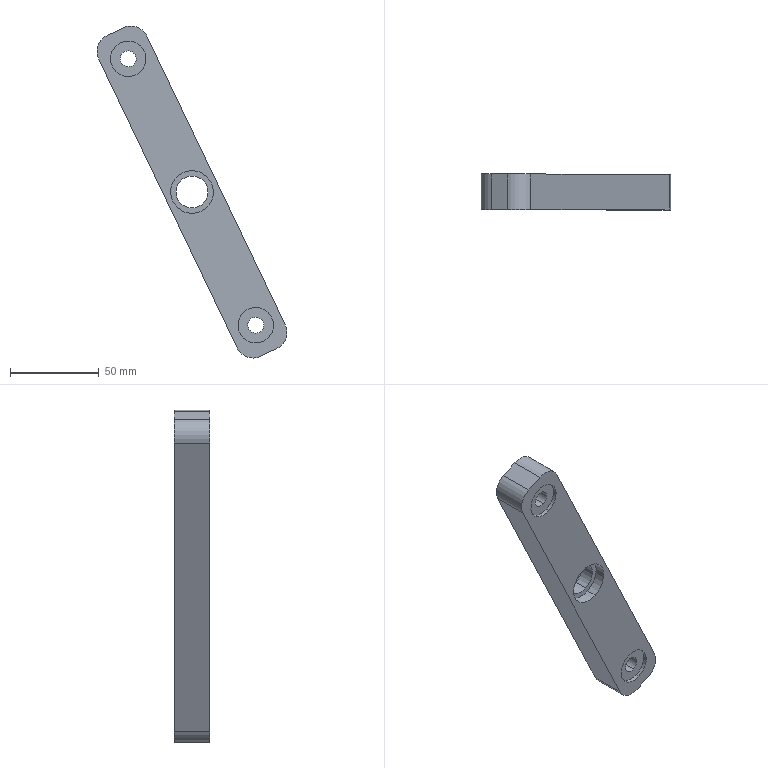Component | SolidWorks | FeedingOpticalAxisFrameConnector1-1-1 | 1 solid | 34 faces | box 106.74 x 20 x 186.67 mm | volume 106028 mm3 | cylinder 22 | plane 12 | commonest cylinder face diameters 20 x8 24 x4 13 x4 9 x4 18 x2
build123d program:
from build123d import *

# Parameters (mm, degrees)
SKETCH1_W                                          = 200
SKETCH1_H                                          = 30
BOSS_EXTRUDE1_DEPTH                                = 20
SKETCH2_R                                          = 10
CUT_EXTRUDE1_DEPTH                                 = 2
HOLE_SIZE_ACCORDING_TO_TYPE_1_OF_HEXAG_D           = 9
HOLE_SIZE_ACCORDING_TO_TYPE_1_OF_HEXAG_CBORE_D     = 13
HOLE_SIZE_ACCORDING_TO_TYPE_1_OF_HEXAG_CBORE_DEPTH = 9
FILLET1_R                                          = 10
F_18_0_18_DIAMETER_HOLE1_D                         = 18
F_18_0_18_DIAMETER_HOLE1_DEPTH                     = 15
F_18_0_18_DIAMETER_HOLE1_TIP                       = 5.408
SKETCH5_R                                          = 12
CUT_EXTRUDE2_DEPTH                                 = 6
CUT_EXTRUDE3_START                                 = -6
SKETCH6_R                                          = 12
CUT_EXTRUDE3_DEPTH                                 = 6


with BuildPart() as part:
    # Sketch1 → Boss-Extrude1 (new body)
    with BuildSketch(Plane.XY):
        with Locations((100, 15)):
            Rectangle(SKETCH1_W, SKETCH1_H)
    extrude(amount=BOSS_EXTRUDE1_DEPTH)

    # Sketch2 → Cut-Extrude1 (cut)
    with BuildSketch(Plane.XY.offset(20)):
        with Locations((17, 15)):
            Circle(SKETCH2_R)
        with Locations((183, 15)):
            Circle(SKETCH2_R)
    extrude(amount=-CUT_EXTRUDE1_DEPTH, mode=Mode.SUBTRACT)

    # Hole Size _According to_ Type 1 of Hexag (through all)
    with Locations(Plane(origin=(17, 15, 0), x_dir=(-1, 0, 0), z_dir=(0, 0, -1))):
        with Locations((0, 0), (-166, 0)):
            CounterBoreHole(HOLE_SIZE_ACCORDING_TO_TYPE_1_OF_HEXAG_D / 2, HOLE_SIZE_ACCORDING_TO_TYPE_1_OF_HEXAG_CBORE_D / 2, HOLE_SIZE_ACCORDING_TO_TYPE_1_OF_HEXAG_CBORE_DEPTH)

    # Fillet1
    fillet1_edges = [part.edges().sort_by_distance(p)[0] for p in [
        (0, 30, 10),
        (200, 30, 10),
        (200, 0, 10),
        (0, 0, 10),
    ]]
    fillet(fillet1_edges, radius=FILLET1_R)

    # 18.0 _18_ Diameter Hole1
    with Locations(Plane(origin=(100, 15, 0), x_dir=(-1, 0, 0), z_dir=(0, 0, -1))):
        with Locations((0, 0)):
            Hole(F_18_0_18_DIAMETER_HOLE1_D / 2, depth=F_18_0_18_DIAMETER_HOLE1_DEPTH)
            with Locations((0, 0, -(F_18_0_18_DIAMETER_HOLE1_DEPTH + F_18_0_18_DIAMETER_HOLE1_TIP / 2))):  # 118° drill point
                Cone(0, F_18_0_18_DIAMETER_HOLE1_D / 2, F_18_0_18_DIAMETER_HOLE1_TIP, mode=Mode.SUBTRACT)

    # Sketch5 → Cut-Extrude2 (cut)
    with BuildSketch(Plane(origin=(0, 0, 0), x_dir=(-1, 0, 0), z_dir=(0, 0, -1))):
        with Locations((-100, 15)):
            Circle(SKETCH5_R)
    extrude(amount=-CUT_EXTRUDE2_DEPTH, mode=Mode.SUBTRACT)

    # Sketch6 → Cut-Extrude3 (cut)
    with BuildSketch(Plane.XY.offset(20).offset(CUT_EXTRUDE3_START)):
        with Locations(Location((100, 15, 0), (0, 0, 180))):
            Circle(SKETCH6_R)
    extrude(amount=CUT_EXTRUDE3_DEPTH, mode=Mode.SUBTRACT)


solid = part.part

# Placed as in the assembly
solid = solid.moved(Location((-51.835, 518, 671.93), (90, 0, -64.419)))
STEP:
#1=CARTESIAN_POINT('',(-0.01214,19.843,23.584));
#2=VERTEX_POINT('',#1);
#3=CARTESIAN_POINT('',(0.3958,19.843,22.732));
#4=VERTEX_POINT('',#3);
#5=CARTESIAN_POINT('',(0.1919,19.843,23.158));
#6=DIRECTION('',(-0.,-1.,-0.));
#7=DIRECTION('',(0.4318,0.,-0.902));
#8=AXIS2_PLACEMENT_3D('',#5,#6,#7);
#9=CIRCLE('',#8,0.4724);
#10=EDGE_CURVE('',#2,#4,#9,.T.);
#11=ORIENTED_EDGE('',*,*,#10,.F.);
#12=CARTESIAN_POINT('',(-0.01214,19.606,23.584));
#13=VERTEX_POINT('',#12);
#14=CARTESIAN_POINT('',(-0.01214,19.843,23.584));
#15=DIRECTION('',(-0.,-1.,-0.));
#16=VECTOR('',#15,39.37);
#17=LINE('',#14,#16);
#18=EDGE_CURVE('',#2,#13,#17,.T.);
#19=ORIENTED_EDGE('',*,*,#18,.T.);
#20=CARTESIAN_POINT('',(0.3958,19.606,22.732));
#21=VERTEX_POINT('',#20);
#22=CARTESIAN_POINT('',(0.1919,19.606,23.158));
#23=DIRECTION('',(-0.,-1.,-0.));
#24=DIRECTION('',(0.4318,0.,-0.902));
#25=AXIS2_PLACEMENT_3D('',#22,#23,#24);
#26=CIRCLE('',#25,0.4724);
#27=EDGE_CURVE('',#13,#21,#26,.T.);
#28=ORIENTED_EDGE('',*,*,#27,.T.);
#29=CARTESIAN_POINT('',(0.3958,19.843,22.732));
#30=DIRECTION('',(-0.,-1.,-0.));
#31=VECTOR('',#30,39.37);
#32=LINE('',#29,#31);
#33=EDGE_CURVE('',#4,#21,#32,.T.);
#34=ORIENTED_EDGE('',*,*,#33,.F.);
#35=EDGE_LOOP('',(#11,#19,#28,#34));
#36=FACE_OUTER_BOUND('',#35,.T.);
#37=CARTESIAN_POINT('',(0.1919,19.843,23.158));
#38=DIRECTION('',(-0.,-1.,-0.));
#39=DIRECTION('',(0.4318,0.,-0.902));
#40=AXIS2_PLACEMENT_3D('',#37,#38,#39);
#41=CYLINDRICAL_SURFACE('',#40,0.4724);
#42=ADVANCED_FACE('',(#36),#41,.F.);
#43=CARTESIAN_POINT('',(0.3958,20.157,22.732));
#44=VERTEX_POINT('',#43);
#45=CARTESIAN_POINT('',(-0.01214,20.157,23.584));
#46=VERTEX_POINT('',#45);
#47=CARTESIAN_POINT('',(0.1919,20.157,23.158));
#48=DIRECTION('',(0.,1.,0.));
#49=DIRECTION('',(-0.4318,0.,0.902));
#50=AXIS2_PLACEMENT_3D('',#47,#48,#49);
#51=CIRCLE('',#50,0.4724);
#52=EDGE_CURVE('',#44,#46,#51,.T.);
#53=ORIENTED_EDGE('',*,*,#52,.F.);
#54=CARTESIAN_POINT('',(0.3958,20.394,22.732));
#55=VERTEX_POINT('',#54);
#56=CARTESIAN_POINT('',(0.3958,20.157,22.732));
#57=DIRECTION('',(0.,1.,0.));
#58=VECTOR('',#57,39.37);
#59=LINE('',#56,#58);
#60=EDGE_CURVE('',#44,#55,#59,.T.);
#61=ORIENTED_EDGE('',*,*,#60,.T.);
#62=CARTESIAN_POINT('',(-0.01214,20.394,23.584));
#63=VERTEX_POINT('',#62);
#64=CARTESIAN_POINT('',(0.1919,20.394,23.158));
#65=DIRECTION('',(0.,1.,0.));
#66=DIRECTION('',(-0.4318,0.,0.902));
#67=AXIS2_PLACEMENT_3D('',#64,#65,#66);
#68=CIRCLE('',#67,0.4724);
#69=EDGE_CURVE('',#55,#63,#68,.T.);
#70=ORIENTED_EDGE('',*,*,#69,.T.);
#71=CARTESIAN_POINT('',(-0.01214,20.157,23.584));
#72=DIRECTION('',(0.,1.,0.));
#73=VECTOR('',#72,39.37);
#74=LINE('',#71,#73);
#75=EDGE_CURVE('',#46,#63,#74,.T.);
#76=ORIENTED_EDGE('',*,*,#75,.F.);
#77=EDGE_LOOP('',(#53,#61,#70,#76));
#78=FACE_OUTER_BOUND('',#77,.T.);
#79=CARTESIAN_POINT('',(0.1919,20.157,23.158));
#80=DIRECTION('',(0.,1.,0.));
#81=DIRECTION('',(-0.4318,0.,0.902));
#82=AXIS2_PLACEMENT_3D('',#79,#80,#81);
#83=CYLINDRICAL_SURFACE('',#82,0.4724);
#84=ADVANCED_FACE('',(#78),#83,.F.);
#85=CARTESIAN_POINT('',(-1.109,20.039,25.874));
#86=VERTEX_POINT('',#85);
#87=CARTESIAN_POINT('',(-1.33,20.039,26.336));
#88=VERTEX_POINT('',#87);
#89=CARTESIAN_POINT('',(-1.219,20.039,26.105));
#90=DIRECTION('',(0.,1.,0.));
#91=DIRECTION('',(-0.4318,0.,0.902));
#92=AXIS2_PLACEMENT_3D('',#89,#90,#91);
#93=CIRCLE('',#92,0.2559);
#94=EDGE_CURVE('',#86,#88,#93,.T.);
#95=ORIENTED_EDGE('',*,*,#94,.F.);
#96=CARTESIAN_POINT('',(-1.109,20.394,25.874));
#97=VERTEX_POINT('',#96);
#98=CARTESIAN_POINT('',(-1.109,20.394,25.874));
#99=DIRECTION('',(0.,1.,0.));
#100=VECTOR('',#99,39.37);
#101=LINE('',#98,#100);
#102=EDGE_CURVE('',#86,#97,#101,.T.);
#103=ORIENTED_EDGE('',*,*,#102,.T.);
#104=CARTESIAN_POINT('',(-1.33,20.394,26.336));
#105=VERTEX_POINT('',#104);
#106=CARTESIAN_POINT('',(-1.219,20.394,26.105));
#107=DIRECTION('',(0.,1.,0.));
#108=DIRECTION('',(-0.4318,0.,0.902));
#109=AXIS2_PLACEMENT_3D('',#106,#107,#108);
#110=CIRCLE('',#109,0.2559);
#111=EDGE_CURVE('',#97,#105,#110,.T.);
#112=ORIENTED_EDGE('',*,*,#111,.T.);
#113=CARTESIAN_POINT('',(-1.33,20.394,26.336));
#114=DIRECTION('',(0.,1.,0.));
#115=VECTOR('',#114,39.37);
#116=LINE('',#113,#115);
#117=EDGE_CURVE('',#88,#105,#116,.T.);
#118=ORIENTED_EDGE('',*,*,#117,.F.);
#119=EDGE_LOOP('',(#95,#103,#112,#118));
#120=FACE_OUTER_BOUND('',#119,.T.);
#121=CARTESIAN_POINT('',(-1.219,20.394,26.105));
#122=DIRECTION('',(0.,1.,0.));
#123=DIRECTION('',(-0.4318,0.,0.902));
#124=AXIS2_PLACEMENT_3D('',#121,#122,#123);
#125=CYLINDRICAL_SURFACE('',#124,0.2559);
#126=ADVANCED_FACE('',(#120),#125,.F.);
#127=CARTESIAN_POINT('',(-1.296,19.685,26.265));
#128=VERTEX_POINT('',#127);
#129=CARTESIAN_POINT('',(-1.143,19.685,25.945));
#130=VERTEX_POINT('',#129);
#131=CARTESIAN_POINT('',(-1.219,19.685,26.105));
#132=DIRECTION('',(-0.,-1.,-0.));
#133=DIRECTION('',(0.4318,0.,-0.902));
#134=AXIS2_PLACEMENT_3D('',#131,#132,#133);
#135=CIRCLE('',#134,0.1772);
#136=EDGE_CURVE('',#128,#130,#135,.T.);
#137=ORIENTED_EDGE('',*,*,#136,.T.);
#138=CARTESIAN_POINT('',(-1.143,20.039,25.945));
#139=VERTEX_POINT('',#138);
#140=CARTESIAN_POINT('',(-1.143,20.394,25.945));
#141=DIRECTION('',(0.,1.,0.));
#142=VECTOR('',#141,39.37);
#143=LINE('',#140,#142);
#144=EDGE_CURVE('',#130,#139,#143,.T.);
#145=ORIENTED_EDGE('',*,*,#144,.T.);
#146=CARTESIAN_POINT('',(-1.296,20.039,26.265));
#147=VERTEX_POINT('',#146);
#148=CARTESIAN_POINT('',(-1.219,20.039,26.105));
#149=DIRECTION('',(0.,1.,0.));
#150=DIRECTION('',(-0.4318,0.,0.902));
#151=AXIS2_PLACEMENT_3D('',#148,#149,#150);
#152=CIRCLE('',#151,0.1772);
#153=EDGE_CURVE('',#139,#147,#152,.T.);
#154=ORIENTED_EDGE('',*,*,#153,.T.);
#155=CARTESIAN_POINT('',(-1.296,20.394,26.265));
#156=DIRECTION('',(0.,1.,0.));
#157=VECTOR('',#156,39.37);
#158=LINE('',#155,#157);
#159=EDGE_CURVE('',#128,#147,#158,.T.);
#160=ORIENTED_EDGE('',*,*,#159,.F.);
#161=EDGE_LOOP('',(#137,#145,#154,#160));
#162=FACE_OUTER_BOUND('',#161,.T.);
#163=CARTESIAN_POINT('',(-1.219,20.394,26.105));
#164=DIRECTION('',(0.,1.,0.));
#165=DIRECTION('',(-0.4318,0.,0.902));
#166=AXIS2_PLACEMENT_3D('',#163,#164,#165);
#167=CYLINDRICAL_SURFACE('',#166,0.1772);
#168=ADVANCED_FACE('',(#162),#167,.F.);
#169=CARTESIAN_POINT('',(1.713,20.039,19.98));
#170=VERTEX_POINT('',#169);
#171=CARTESIAN_POINT('',(1.492,20.039,20.441));
#172=VERTEX_POINT('',#171);
#173=CARTESIAN_POINT('',(1.603,20.039,20.21));
#174=DIRECTION('',(0.,1.,0.));
#175=DIRECTION('',(-0.4318,0.,0.902));
#176=AXIS2_PLACEMENT_3D('',#173,#174,#175);
#177=CIRCLE('',#176,0.2559);
#178=EDGE_CURVE('',#170,#172,#177,.T.);
#179=ORIENTED_EDGE('',*,*,#178,.F.);
#180=CARTESIAN_POINT('',(1.713,20.394,19.98));
#181=VERTEX_POINT('',#180);
#182=CARTESIAN_POINT('',(1.713,20.394,19.98));
#183=DIRECTION('',(0.,1.,0.));
#184=VECTOR('',#183,39.37);
#185=LINE('',#182,#184);
#186=EDGE_CURVE('',#170,#181,#185,.T.);
#187=ORIENTED_EDGE('',*,*,#186,.T.);
#188=CARTESIAN_POINT('',(1.492,20.394,20.441));
#189=VERTEX_POINT('',#188);
#190=CARTESIAN_POINT('',(1.603,20.394,20.21));
#191=DIRECTION('',(0.,1.,0.));
#192=DIRECTION('',(-0.4318,0.,0.902));
#193=AXIS2_PLACEMENT_3D('',#190,#191,#192);
#194=CIRCLE('',#193,0.2559);
#195=EDGE_CURVE('',#181,#189,#194,.T.);
#196=ORIENTED_EDGE('',*,*,#195,.T.);
#197=CARTESIAN_POINT('',(1.492,20.394,20.441));
#198=DIRECTION('',(0.,1.,0.));
#199=VECTOR('',#198,39.37);
#200=LINE('',#197,#199);
#201=EDGE_CURVE('',#172,#189,#200,.T.);
#202=ORIENTED_EDGE('',*,*,#201,.F.);
#203=EDGE_LOOP('',(#179,#187,#196,#202));
#204=FACE_OUTER_BOUND('',#203,.T.);
#205=CARTESIAN_POINT('',(1.603,20.394,20.21));
#206=DIRECTION('',(0.,1.,0.));
#207=DIRECTION('',(-0.4318,0.,0.902));
#208=AXIS2_PLACEMENT_3D('',#205,#206,#207);
#209=CYLINDRICAL_SURFACE('',#208,0.2559);
#210=ADVANCED_FACE('',(#204),#209,.F.);
#211=CARTESIAN_POINT('',(1.526,19.685,20.37));
#212=VERTEX_POINT('',#211);
#213=CARTESIAN_POINT('',(1.679,19.685,20.051));
#214=VERTEX_POINT('',#213);
#215=CARTESIAN_POINT('',(1.603,19.685,20.21));
#216=DIRECTION('',(-0.,-1.,-0.));
#217=DIRECTION('',(0.4318,0.,-0.902));
#218=AXIS2_PLACEMENT_3D('',#215,#216,#217);
#219=CIRCLE('',#218,0.1772);
#220=EDGE_CURVE('',#212,#214,#219,.T.);
#221=ORIENTED_EDGE('',*,*,#220,.T.);
#222=CARTESIAN_POINT('',(1.679,20.039,20.051));
#223=VERTEX_POINT('',#222);
#224=CARTESIAN_POINT('',(1.679,20.394,20.051));
#225=DIRECTION('',(0.,1.,0.));
#226=VECTOR('',#225,39.37);
#227=LINE('',#224,#226);
#228=EDGE_CURVE('',#214,#223,#227,.T.);
#229=ORIENTED_EDGE('',*,*,#228,.T.);
#230=CARTESIAN_POINT('',(1.526,20.039,20.37));
#231=VERTEX_POINT('',#230);
#232=CARTESIAN_POINT('',(1.603,20.039,20.21));
#233=DIRECTION('',(0.,1.,0.));
#234=DIRECTION('',(-0.4318,0.,0.902));
#235=AXIS2_PLACEMENT_3D('',#232,#233,#234);
#236=CIRCLE('',#235,0.1772);
#237=EDGE_CURVE('',#223,#231,#236,.T.);
#238=ORIENTED_EDGE('',*,*,#237,.T.);
#239=CARTESIAN_POINT('',(1.526,20.394,20.37));
#240=DIRECTION('',(0.,1.,0.));
#241=VECTOR('',#240,39.37);
#242=LINE('',#239,#241);
#243=EDGE_CURVE('',#212,#231,#242,.T.);
#244=ORIENTED_EDGE('',*,*,#243,.F.);
#245=EDGE_LOOP('',(#221,#229,#238,#244));
#246=FACE_OUTER_BOUND('',#245,.T.);
#247=CARTESIAN_POINT('',(1.603,20.394,20.21));
#248=DIRECTION('',(0.,1.,0.));
#249=DIRECTION('',(-0.4318,0.,0.902));
#250=AXIS2_PLACEMENT_3D('',#247,#248,#249);
#251=CYLINDRICAL_SURFACE('',#250,0.1772);
#252=ADVANCED_FACE('',(#246),#251,.F.);
#253=CARTESIAN_POINT('',(1.433,19.685,20.566));
#254=VERTEX_POINT('',#253);
#255=CARTESIAN_POINT('',(1.773,19.685,19.855));
#256=VERTEX_POINT('',#255);
#257=CARTESIAN_POINT('',(1.603,19.685,20.21));
#258=DIRECTION('',(-0.,-1.,-0.));
#259=DIRECTION('',(0.4318,0.,-0.902));
#260=AXIS2_PLACEMENT_3D('',#257,#258,#259);
#261=CIRCLE('',#260,0.3937);
#262=EDGE_CURVE('',#254,#256,#261,.T.);
#263=ORIENTED_EDGE('',*,*,#262,.F.);
#264=CARTESIAN_POINT('',(1.433,19.606,20.566));
#265=VERTEX_POINT('',#264);
#266=CARTESIAN_POINT('',(1.433,19.685,20.566));
#267=DIRECTION('',(-0.,-1.,-0.));
#268=VECTOR('',#267,39.37);
#269=LINE('',#266,#268);
#270=EDGE_CURVE('',#254,#265,#269,.T.);
#271=ORIENTED_EDGE('',*,*,#270,.T.);
#272=CARTESIAN_POINT('',(1.773,19.606,19.855));
#273=VERTEX_POINT('',#272);
#274=CARTESIAN_POINT('',(1.603,19.606,20.21));
#275=DIRECTION('',(-0.,-1.,-0.));
#276=DIRECTION('',(0.4318,0.,-0.902));
#277=AXIS2_PLACEMENT_3D('',#274,#275,#276);
#278=CIRCLE('',#277,0.3937);
#279=EDGE_CURVE('',#265,#273,#278,.T.);
#280=ORIENTED_EDGE('',*,*,#279,.T.);
#281=CARTESIAN_POINT('',(1.773,19.685,19.855));
#282=DIRECTION('',(-0.,-1.,-0.));
#283=VECTOR('',#282,39.37);
#284=LINE('',#281,#283);
#285=EDGE_CURVE('',#256,#273,#284,.T.);
#286=ORIENTED_EDGE('',*,*,#285,.F.);
#287=EDGE_LOOP('',(#263,#271,#280,#286));
#288=FACE_OUTER_BOUND('',#287,.T.);
#289=CARTESIAN_POINT('',(1.603,19.685,20.21));
#290=DIRECTION('',(-0.,-1.,-0.));
#291=DIRECTION('',(0.4318,0.,-0.902));
#292=AXIS2_PLACEMENT_3D('',#289,#290,#291);
#293=CYLINDRICAL_SURFACE('',#292,0.3937);
#294=ADVANCED_FACE('',(#288),#293,.F.);
#295=CARTESIAN_POINT('',(-1.389,19.685,26.46));
#296=VERTEX_POINT('',#295);
#297=CARTESIAN_POINT('',(-1.049,19.685,25.75));
#298=VERTEX_POINT('',#297);
#299=CARTESIAN_POINT('',(-1.219,19.685,26.105));
#300=DIRECTION('',(-0.,-1.,-0.));
#301=DIRECTION('',(0.4318,0.,-0.902));
#302=AXIS2_PLACEMENT_3D('',#299,#300,#301);
#303=CIRCLE('',#302,0.3937);
#304=EDGE_CURVE('',#296,#298,#303,.T.);
#305=ORIENTED_EDGE('',*,*,#304,.F.);
#306=CARTESIAN_POINT('',(-1.389,19.606,26.46));
#307=VERTEX_POINT('',#306);
#308=CARTESIAN_POINT('',(-1.389,19.685,26.46));
#309=DIRECTION('',(-0.,-1.,-0.));
#310=VECTOR('',#309,39.37);
#311=LINE('',#308,#310);
#312=EDGE_CURVE('',#296,#307,#311,.T.);
#313=ORIENTED_EDGE('',*,*,#312,.T.);
#314=CARTESIAN_POINT('',(-1.049,19.606,25.75));
#315=VERTEX_POINT('',#314);
#316=CARTESIAN_POINT('',(-1.219,19.606,26.105));
#317=DIRECTION('',(-0.,-1.,-0.));
#318=DIRECTION('',(0.4318,0.,-0.902));
#319=AXIS2_PLACEMENT_3D('',#316,#317,#318);
#320=CIRCLE('',#319,0.3937);
#321=EDGE_CURVE('',#307,#315,#320,.T.);
#322=ORIENTED_EDGE('',*,*,#321,.T.);
#323=CARTESIAN_POINT('',(-1.049,19.685,25.75));
#324=DIRECTION('',(-0.,-1.,-0.));
#325=VECTOR('',#324,39.37);
#326=LINE('',#323,#325);
#327=EDGE_CURVE('',#298,#315,#326,.T.);
#328=ORIENTED_EDGE('',*,*,#327,.F.);
#329=EDGE_LOOP('',(#305,#313,#322,#328));
#330=FACE_OUTER_BOUND('',#329,.T.);
#331=CARTESIAN_POINT('',(-1.219,19.685,26.105));
#332=DIRECTION('',(-0.,-1.,-0.));
#333=DIRECTION('',(0.4318,0.,-0.902));
#334=AXIS2_PLACEMENT_3D('',#331,#332,#333);
#335=CYLINDRICAL_SURFACE('',#334,0.3937);
#336=ADVANCED_FACE('',(#330),#335,.F.);
#337=CARTESIAN_POINT('',(0.3449,19.843,22.838));
#338=VERTEX_POINT('',#337);
#339=CARTESIAN_POINT('',(0.03886,19.843,23.477));
#340=VERTEX_POINT('',#339);
#341=CARTESIAN_POINT('',(0.1919,19.843,23.158));
#342=DIRECTION('',(0.,1.,0.));
#343=DIRECTION('',(0.4318,0.,-0.902));
#344=AXIS2_PLACEMENT_3D('',#341,#342,#343);
#345=CIRCLE('',#344,0.3543);
#346=EDGE_CURVE('',#338,#340,#345,.T.);
#347=ORIENTED_EDGE('',*,*,#346,.F.);
#348=CARTESIAN_POINT('',(0.3449,20.157,22.838));
#349=VERTEX_POINT('',#348);
#350=CARTESIAN_POINT('',(0.3449,20.394,22.838));
#351=DIRECTION('',(0.,1.,0.));
#352=VECTOR('',#351,39.37);
#353=LINE('',#350,#352);
#354=EDGE_CURVE('',#338,#349,#353,.T.);
#355=ORIENTED_EDGE('',*,*,#354,.T.);
#356=CARTESIAN_POINT('',(0.03886,20.157,23.477));
#357=VERTEX_POINT('',#356);
#358=CARTESIAN_POINT('',(0.1919,20.157,23.158));
#359=DIRECTION('',(-0.,-1.,-0.));
#360=DIRECTION('',(-0.4318,0.,0.902));
#361=AXIS2_PLACEMENT_3D('',#358,#359,#360);
#362=CIRCLE('',#361,0.3543);
#363=EDGE_CURVE('',#357,#349,#362,.T.);
#364=ORIENTED_EDGE('',*,*,#363,.F.);
#365=CARTESIAN_POINT('',(0.03886,20.394,23.477));
#366=DIRECTION('',(0.,1.,0.));
#367=VECTOR('',#366,39.37);
#368=LINE('',#365,#367);
#369=EDGE_CURVE('',#340,#357,#368,.T.);
#370=ORIENTED_EDGE('',*,*,#369,.F.);
#371=EDGE_LOOP('',(#347,#355,#364,#370));
#372=FACE_OUTER_BOUND('',#371,.T.);
#373=CARTESIAN_POINT('',(0.1919,20.394,23.158));
#374=DIRECTION('',(0.,1.,0.));
#375=DIRECTION('',(-0.4318,0.,0.902));
#376=AXIS2_PLACEMENT_3D('',#373,#374,#375);
#377=CYLINDRICAL_SURFACE('',#376,0.3543);
#378=ADVANCED_FACE('',(#372),#377,.F.);
#379=ORIENTED_EDGE('',*,*,#354,.F.);
#380=CARTESIAN_POINT('',(0.1919,19.843,23.158));
#381=DIRECTION('',(0.,1.,0.));
#382=DIRECTION('',(0.4318,0.,-0.902));
#383=AXIS2_PLACEMENT_3D('',#380,#381,#382);
#384=CIRCLE('',#383,0.3543);
#385=EDGE_CURVE('',#340,#338,#384,.T.);
#386=ORIENTED_EDGE('',*,*,#385,.F.);
#387=ORIENTED_EDGE('',*,*,#369,.T.);
#388=CARTESIAN_POINT('',(0.1919,20.157,23.158));
#389=DIRECTION('',(-0.,-1.,-0.));
#390=DIRECTION('',(-0.4318,0.,0.902));
#391=AXIS2_PLACEMENT_3D('',#388,#389,#390);
#392=CIRCLE('',#391,0.3543);
#393=EDGE_CURVE('',#349,#357,#392,.T.);
#394=ORIENTED_EDGE('',*,*,#393,.F.);
#395=EDGE_LOOP('',(#379,#386,#387,#394));
#396=FACE_OUTER_BOUND('',#395,.T.);
#397=CARTESIAN_POINT('',(0.1919,20.394,23.158));
#398=DIRECTION('',(0.,1.,0.));
#399=DIRECTION('',(-0.4318,0.,0.902));
#400=AXIS2_PLACEMENT_3D('',#397,#398,#399);
#401=CYLINDRICAL_SURFACE('',#400,0.3543);
#402=ADVANCED_FACE('',(#396),#401,.F.);
#403=CARTESIAN_POINT('',(-1.331,20.394,26.794));
#404=VERTEX_POINT('',#403);
#405=CARTESIAN_POINT('',(-1.686,20.394,26.624));
#406=VERTEX_POINT('',#405);
#407=CARTESIAN_POINT('',(-2.041,20.394,26.454));
#408=DIRECTION('',(-0.902,0.,-0.4318));
#409=VECTOR('',#408,39.37);
#410=LINE('',#407,#409);
#411=EDGE_CURVE('',#404,#406,#410,.T.);
#412=ORIENTED_EDGE('',*,*,#411,.T.);
#413=CARTESIAN_POINT('',(-1.686,19.606,26.624));
#414=VERTEX_POINT('',#413);
#415=CARTESIAN_POINT('',(-1.686,19.606,26.624));
#416=DIRECTION('',(-0.,-1.,-0.));
#417=VECTOR('',#416,39.37);
#418=LINE('',#415,#417);
#419=EDGE_CURVE('',#406,#414,#418,.T.);
#420=ORIENTED_EDGE('',*,*,#419,.T.);
#421=CARTESIAN_POINT('',(-1.331,19.606,26.794));
#422=VERTEX_POINT('',#421);
#423=CARTESIAN_POINT('',(-2.041,19.606,26.454));
#424=DIRECTION('',(-0.902,0.,-0.4318));
#425=VECTOR('',#424,39.37);
#426=LINE('',#423,#425);
#427=EDGE_CURVE('',#422,#414,#426,.T.);
#428=ORIENTED_EDGE('',*,*,#427,.F.);
#429=CARTESIAN_POINT('',(-1.331,19.606,26.794));
#430=DIRECTION('',(0.,1.,0.));
#431=VECTOR('',#430,39.37);
#432=LINE('',#429,#431);
#433=EDGE_CURVE('',#422,#404,#432,.T.);
#434=ORIENTED_EDGE('',*,*,#433,.T.);
#435=EDGE_LOOP('',(#412,#420,#428,#434));
#436=FACE_OUTER_BOUND('',#435,.T.);
#437=CARTESIAN_POINT('',(-2.041,19.606,26.454));
#438=DIRECTION('',(0.4318,-0.,-0.902));
#439=DIRECTION('',(0.,1.,0.));
#440=AXIS2_PLACEMENT_3D('',#437,#438,#439);
#441=PLANE('',#440);
#442=ADVANCED_FACE('',(#436),#441,.F.);
#443=CARTESIAN_POINT('',(-1.871,19.606,26.099));
#444=VERTEX_POINT('',#443);
#445=CARTESIAN_POINT('',(1.189,19.606,19.707));
#446=VERTEX_POINT('',#445);
#447=CARTESIAN_POINT('',(-2.041,19.606,26.454));
#448=DIRECTION('',(0.4318,-0.,-0.902));
#449=VECTOR('',#448,39.37);
#450=LINE('',#447,#449);
#451=EDGE_CURVE('',#444,#446,#450,.T.);
#452=ORIENTED_EDGE('',*,*,#451,.F.);
#453=CARTESIAN_POINT('',(-1.871,20.394,26.099));
#454=VERTEX_POINT('',#453);
#455=CARTESIAN_POINT('',(-1.871,19.606,26.099));
#456=DIRECTION('',(0.,1.,0.));
#457=VECTOR('',#456,39.37);
#458=LINE('',#455,#457);
#459=EDGE_CURVE('',#444,#454,#458,.T.);
#460=ORIENTED_EDGE('',*,*,#459,.T.);
#461=CARTESIAN_POINT('',(1.189,20.394,19.707));
#462=VERTEX_POINT('',#461);
#463=CARTESIAN_POINT('',(-2.041,20.394,26.454));
#464=DIRECTION('',(0.4318,-0.,-0.902));
#465=VECTOR('',#464,39.37);
#466=LINE('',#463,#465);
#467=EDGE_CURVE('',#454,#462,#466,.T.);
#468=ORIENTED_EDGE('',*,*,#467,.T.);
#469=CARTESIAN_POINT('',(1.189,19.606,19.707));
#470=DIRECTION('',(-0.,-1.,-0.));
#471=VECTOR('',#470,39.37);
#472=LINE('',#469,#471);
#473=EDGE_CURVE('',#462,#446,#472,.T.);
#474=ORIENTED_EDGE('',*,*,#473,.T.);
#475=EDGE_LOOP('',(#452,#460,#468,#474));
#476=FACE_OUTER_BOUND('',#475,.T.);
#477=CARTESIAN_POINT('',(-2.041,19.606,26.454));
#478=DIRECTION('',(0.902,-0.,0.4318));
#479=DIRECTION('',(-0.,-1.,-0.));
#480=AXIS2_PLACEMENT_3D('',#477,#478,#479);
#481=PLANE('',#480);
#482=ADVANCED_FACE('',(#476),#481,.F.);
#483=CARTESIAN_POINT('',(1.714,19.606,19.522));
#484=VERTEX_POINT('',#483);
#485=CARTESIAN_POINT('',(2.069,19.606,19.692));
#486=VERTEX_POINT('',#485);
#487=CARTESIAN_POINT('',(1.359,19.606,19.352));
#488=DIRECTION('',(0.902,-0.,0.4318));
#489=VECTOR('',#488,39.37);
#490=LINE('',#487,#489);
#491=EDGE_CURVE('',#484,#486,#490,.T.);
#492=ORIENTED_EDGE('',*,*,#491,.F.);
#493=CARTESIAN_POINT('',(1.714,20.394,19.522));
#494=VERTEX_POINT('',#493);
#495=CARTESIAN_POINT('',(1.714,19.606,19.522));
#496=DIRECTION('',(0.,1.,0.));
#497=VECTOR('',#496,39.37);
#498=LINE('',#495,#497);
#499=EDGE_CURVE('',#484,#494,#498,.T.);
#500=ORIENTED_EDGE('',*,*,#499,.T.);
#501=CARTESIAN_POINT('',(2.069,20.394,19.692));
#502=VERTEX_POINT('',#501);
#503=CARTESIAN_POINT('',(1.359,20.394,19.352));
#504=DIRECTION('',(0.902,-0.,0.4318));
#505=VECTOR('',#504,39.37);
#506=LINE('',#503,#505);
#507=EDGE_CURVE('',#494,#502,#506,.T.);
#508=ORIENTED_EDGE('',*,*,#507,.T.);
#509=CARTESIAN_POINT('',(2.069,19.606,19.692));
#510=DIRECTION('',(-0.,-1.,-0.));
#511=VECTOR('',#510,39.37);
#512=LINE('',#509,#511);
#513=EDGE_CURVE('',#502,#486,#512,.T.);
#514=ORIENTED_EDGE('',*,*,#513,.T.);
#515=EDGE_LOOP('',(#492,#500,#508,#514));
#516=FACE_OUTER_BOUND('',#515,.T.);
#517=CARTESIAN_POINT('',(1.359,19.606,19.352));
#518=DIRECTION('',(-0.4318,0.,0.902));
#519=DIRECTION('',(-0.,-1.,-0.));
#520=AXIS2_PLACEMENT_3D('',#517,#518,#519);
#521=PLANE('',#520);
#522=ADVANCED_FACE('',(#516),#521,.F.);
#523=CARTESIAN_POINT('',(2.254,20.394,20.217));
#524=VERTEX_POINT('',#523);
#525=CARTESIAN_POINT('',(-0.8054,20.394,26.609));
#526=VERTEX_POINT('',#525);
#527=CARTESIAN_POINT('',(-0.9754,20.394,26.964));
#528=DIRECTION('',(-0.4318,0.,0.902));
#529=VECTOR('',#528,39.37);
#530=LINE('',#527,#529);
#531=EDGE_CURVE('',#524,#526,#530,.T.);
#532=ORIENTED_EDGE('',*,*,#531,.T.);
#533=CARTESIAN_POINT('',(-0.8054,19.606,26.609));
#534=VERTEX_POINT('',#533);
#535=CARTESIAN_POINT('',(-0.8054,19.606,26.609));
#536=DIRECTION('',(-0.,-1.,-0.));
#537=VECTOR('',#536,39.37);
#538=LINE('',#535,#537);
#539=EDGE_CURVE('',#526,#534,#538,.T.);
#540=ORIENTED_EDGE('',*,*,#539,.T.);
#541=CARTESIAN_POINT('',(2.254,19.606,20.217));
#542=VERTEX_POINT('',#541);
#543=CARTESIAN_POINT('',(-0.9754,19.606,26.964));
#544=DIRECTION('',(-0.4318,0.,0.902));
#545=VECTOR('',#544,39.37);
#546=LINE('',#543,#545);
#547=EDGE_CURVE('',#542,#534,#546,.T.);
#548=ORIENTED_EDGE('',*,*,#547,.F.);
#549=CARTESIAN_POINT('',(2.254,19.606,20.217));
#550=DIRECTION('',(0.,1.,0.));
#551=VECTOR('',#550,39.37);
#552=LINE('',#549,#551);
#553=EDGE_CURVE('',#542,#524,#552,.T.);
#554=ORIENTED_EDGE('',*,*,#553,.T.);
#555=EDGE_LOOP('',(#532,#540,#548,#554));
#556=FACE_OUTER_BOUND('',#555,.T.);
#557=CARTESIAN_POINT('',(-0.9754,19.606,26.964));
#558=DIRECTION('',(-0.902,0.,-0.4318));
#559=DIRECTION('',(0.,1.,0.));
#560=AXIS2_PLACEMENT_3D('',#557,#558,#559);
#561=PLANE('',#560);
#562=ADVANCED_FACE('',(#556),#561,.F.);
#563=CARTESIAN_POINT('',(0.1919,19.606,23.158));
#564=DIRECTION('',(-0.,-1.,-0.));
#565=DIRECTION('',(0.4318,0.,-0.902));
#566=AXIS2_PLACEMENT_3D('',#563,#564,#565);
#567=CIRCLE('',#566,0.4724);
#568=EDGE_CURVE('',#21,#13,#567,.T.);
#569=ORIENTED_EDGE('',*,*,#568,.F.);
#570=ORIENTED_EDGE('',*,*,#27,.F.);
#571=EDGE_LOOP('',(#569,#570));
#572=FACE_BOUND('',#571,.T.);
#573=CARTESIAN_POINT('',(1.603,19.606,20.21));
#574=DIRECTION('',(-0.,-1.,-0.));
#575=DIRECTION('',(0.4318,0.,-0.902));
#576=AXIS2_PLACEMENT_3D('',#573,#574,#575);
#577=CIRCLE('',#576,0.3937);
#578=EDGE_CURVE('',#273,#265,#577,.T.);
#579=ORIENTED_EDGE('',*,*,#578,.F.);
#580=ORIENTED_EDGE('',*,*,#279,.F.);
#581=EDGE_LOOP('',(#579,#580));
#582=FACE_BOUND('',#581,.T.);
#583=CARTESIAN_POINT('',(-1.219,19.606,26.105));
#584=DIRECTION('',(-0.,-1.,-0.));
#585=DIRECTION('',(0.4318,0.,-0.902));
#586=AXIS2_PLACEMENT_3D('',#583,#584,#585);
#587=CIRCLE('',#586,0.3937);
#588=EDGE_CURVE('',#315,#307,#587,.T.);
#589=ORIENTED_EDGE('',*,*,#588,.F.);
#590=ORIENTED_EDGE('',*,*,#321,.F.);
#591=EDGE_LOOP('',(#589,#590));
#592=FACE_BOUND('',#591,.T.);
#593=ORIENTED_EDGE('',*,*,#427,.T.);
#594=CARTESIAN_POINT('',(-1.516,19.606,26.269));
#595=DIRECTION('',(-0.,-1.,-0.));
#596=DIRECTION('',(-0.4318,0.,0.902));
#597=AXIS2_PLACEMENT_3D('',#594,#595,#596);
#598=CIRCLE('',#597,0.3937);
#599=EDGE_CURVE('',#414,#444,#598,.T.);
#600=ORIENTED_EDGE('',*,*,#599,.T.);
#601=ORIENTED_EDGE('',*,*,#451,.T.);
#602=CARTESIAN_POINT('',(1.544,19.606,19.877));
#603=DIRECTION('',(-0.,-1.,-0.));
#604=DIRECTION('',(-0.4318,0.,0.902));
#605=AXIS2_PLACEMENT_3D('',#602,#603,#604);
#606=CIRCLE('',#605,0.3937);
#607=EDGE_CURVE('',#446,#484,#606,.T.);
#608=ORIENTED_EDGE('',*,*,#607,.T.);
#609=ORIENTED_EDGE('',*,*,#491,.T.);
#610=CARTESIAN_POINT('',(1.899,19.606,20.047));
#611=DIRECTION('',(-0.,-1.,-0.));
#612=DIRECTION('',(-0.4318,0.,0.902));
#613=AXIS2_PLACEMENT_3D('',#610,#611,#612);
#614=CIRCLE('',#613,0.3937);
#615=EDGE_CURVE('',#486,#542,#614,.T.);
#616=ORIENTED_EDGE('',*,*,#615,.T.);
#617=ORIENTED_EDGE('',*,*,#547,.T.);
#618=CARTESIAN_POINT('',(-1.161,19.606,26.439));
#619=DIRECTION('',(-0.,-1.,-0.));
#620=DIRECTION('',(-0.4318,0.,0.902));
#621=AXIS2_PLACEMENT_3D('',#618,#619,#620);
#622=CIRCLE('',#621,0.3937);
#623=EDGE_CURVE('',#534,#422,#622,.T.);
#624=ORIENTED_EDGE('',*,*,#623,.T.);
#625=EDGE_LOOP('',(#593,#600,#601,#608,#609,#616,#617,#624));
#626=FACE_OUTER_BOUND('',#625,.T.);
#627=CARTESIAN_POINT('',(-2.041,19.606,26.454));
#628=DIRECTION('',(0.,1.,0.));
#629=DIRECTION('',(-0.4318,0.,0.902));
#630=AXIS2_PLACEMENT_3D('',#627,#628,#629);
#631=PLANE('',#630);
#632=ADVANCED_FACE('',(#572,#582,#592,#626),#631,.F.);
#633=CARTESIAN_POINT('',(0.1919,20.394,23.158));
#634=DIRECTION('',(0.,1.,0.));
#635=DIRECTION('',(-0.4318,0.,0.902));
#636=AXIS2_PLACEMENT_3D('',#633,#634,#635);
#637=CIRCLE('',#636,0.4724);
#638=EDGE_CURVE('',#63,#55,#637,.T.);
#639=ORIENTED_EDGE('',*,*,#638,.F.);
#640=ORIENTED_EDGE('',*,*,#69,.F.);
#641=EDGE_LOOP('',(#639,#640));
#642=FACE_BOUND('',#641,.T.);
#643=CARTESIAN_POINT('',(-1.219,20.394,26.105));
#644=DIRECTION('',(0.,1.,0.));
#645=DIRECTION('',(-0.4318,0.,0.902));
#646=AXIS2_PLACEMENT_3D('',#643,#644,#645);
#647=CIRCLE('',#646,0.2559);
#648=EDGE_CURVE('',#105,#97,#647,.T.);
#649=ORIENTED_EDGE('',*,*,#648,.F.);
#650=ORIENTED_EDGE('',*,*,#111,.F.);
#651=EDGE_LOOP('',(#649,#650));
#652=FACE_BOUND('',#651,.T.);
#653=CARTESIAN_POINT('',(1.603,20.394,20.21));
#654=DIRECTION('',(0.,1.,0.));
#655=DIRECTION('',(-0.4318,0.,0.902));
#656=AXIS2_PLACEMENT_3D('',#653,#654,#655);
#657=CIRCLE('',#656,0.2559);
#658=EDGE_CURVE('',#189,#181,#657,.T.);
#659=ORIENTED_EDGE('',*,*,#658,.F.);
#660=ORIENTED_EDGE('',*,*,#195,.F.);
#661=EDGE_LOOP('',(#659,#660));
#662=FACE_BOUND('',#661,.T.);
#663=ORIENTED_EDGE('',*,*,#467,.F.);
#664=CARTESIAN_POINT('',(-1.516,20.394,26.269));
#665=DIRECTION('',(0.,1.,0.));
#666=DIRECTION('',(-0.4318,0.,0.902));
#667=AXIS2_PLACEMENT_3D('',#664,#665,#666);
#668=CIRCLE('',#667,0.3937);
#669=EDGE_CURVE('',#454,#406,#668,.T.);
#670=ORIENTED_EDGE('',*,*,#669,.T.);
#671=ORIENTED_EDGE('',*,*,#411,.F.);
#672=CARTESIAN_POINT('',(-1.161,20.394,26.439));
#673=DIRECTION('',(0.,1.,0.));
#674=DIRECTION('',(-0.4318,0.,0.902));
#675=AXIS2_PLACEMENT_3D('',#672,#673,#674);
#676=CIRCLE('',#675,0.3937);
#677=EDGE_CURVE('',#404,#526,#676,.T.);
#678=ORIENTED_EDGE('',*,*,#677,.T.);
#679=ORIENTED_EDGE('',*,*,#531,.F.);
#680=CARTESIAN_POINT('',(1.899,20.394,20.047));
#681=DIRECTION('',(0.,1.,0.));
#682=DIRECTION('',(-0.4318,0.,0.902));
#683=AXIS2_PLACEMENT_3D('',#680,#681,#682);
#684=CIRCLE('',#683,0.3937);
#685=EDGE_CURVE('',#524,#502,#684,.T.);
#686=ORIENTED_EDGE('',*,*,#685,.T.);
#687=ORIENTED_EDGE('',*,*,#507,.F.);
#688=CARTESIAN_POINT('',(1.544,20.394,19.877));
#689=DIRECTION('',(0.,1.,0.));
#690=DIRECTION('',(-0.4318,0.,0.902));
#691=AXIS2_PLACEMENT_3D('',#688,#689,#690);
#692=CIRCLE('',#691,0.3937);
#693=EDGE_CURVE('',#494,#462,#692,.T.);
#694=ORIENTED_EDGE('',*,*,#693,.T.);
#695=EDGE_LOOP('',(#663,#670,#671,#678,#679,#686,#687,#694));
#696=FACE_OUTER_BOUND('',#695,.T.);
#697=CARTESIAN_POINT('',(-2.041,20.394,26.454));
#698=DIRECTION('',(0.,1.,0.));
#699=DIRECTION('',(-0.4318,0.,0.902));
#700=AXIS2_PLACEMENT_3D('',#697,#698,#699);
#701=PLANE('',#700);
#702=ADVANCED_FACE('',(#642,#652,#662,#696),#701,.T.);
#703=ORIENTED_EDGE('',*,*,#312,.F.);
#704=CARTESIAN_POINT('',(-1.219,19.685,26.105));
#705=DIRECTION('',(-0.,-1.,-0.));
#706=DIRECTION('',(0.4318,0.,-0.902));
#707=AXIS2_PLACEMENT_3D('',#704,#705,#706);
#708=CIRCLE('',#707,0.3937);
#709=EDGE_CURVE('',#298,#296,#708,.T.);
#710=ORIENTED_EDGE('',*,*,#709,.F.);
#711=ORIENTED_EDGE('',*,*,#327,.T.);
#712=ORIENTED_EDGE('',*,*,#588,.T.);
#713=EDGE_LOOP('',(#703,#710,#711,#712));
#714=FACE_OUTER_BOUND('',#713,.T.);
#715=CARTESIAN_POINT('',(-1.219,19.685,26.105));
#716=DIRECTION('',(-0.,-1.,-0.));
#717=DIRECTION('',(0.4318,0.,-0.902));
#718=AXIS2_PLACEMENT_3D('',#715,#716,#717);
#719=CYLINDRICAL_SURFACE('',#718,0.3937);
#720=ADVANCED_FACE('',(#714),#719,.F.);
#721=ORIENTED_EDGE('',*,*,#136,.F.);
#722=CARTESIAN_POINT('',(-1.219,19.685,26.105));
#723=DIRECTION('',(-0.,-1.,-0.));
#724=DIRECTION('',(0.4318,0.,-0.902));
#725=AXIS2_PLACEMENT_3D('',#722,#723,#724);
#726=CIRCLE('',#725,0.1772);
#727=EDGE_CURVE('',#130,#128,#726,.T.);
#728=ORIENTED_EDGE('',*,*,#727,.F.);
#729=EDGE_LOOP('',(#721,#728));
#730=FACE_BOUND('',#729,.T.);
#731=ORIENTED_EDGE('',*,*,#709,.T.);
#732=ORIENTED_EDGE('',*,*,#304,.T.);
#733=EDGE_LOOP('',(#731,#732));
#734=FACE_OUTER_BOUND('',#733,.T.);
#735=CARTESIAN_POINT('',(-1.219,19.685,26.105));
#736=DIRECTION('',(-0.,-1.,-0.));
#737=DIRECTION('',(0.4318,-0.,-0.902));
#738=AXIS2_PLACEMENT_3D('',#735,#736,#737);
#739=PLANE('',#738);
#740=ADVANCED_FACE('',(#730,#734),#739,.T.);
#741=ORIENTED_EDGE('',*,*,#270,.F.);
#742=CARTESIAN_POINT('',(1.603,19.685,20.21));
#743=DIRECTION('',(-0.,-1.,-0.));
#744=DIRECTION('',(0.4318,0.,-0.902));
#745=AXIS2_PLACEMENT_3D('',#742,#743,#744);
#746=CIRCLE('',#745,0.3937);
#747=EDGE_CURVE('',#256,#254,#746,.T.);
#748=ORIENTED_EDGE('',*,*,#747,.F.);
#749=ORIENTED_EDGE('',*,*,#285,.T.);
#750=ORIENTED_EDGE('',*,*,#578,.T.);
#751=EDGE_LOOP('',(#741,#748,#749,#750));
#752=FACE_OUTER_BOUND('',#751,.T.);
#753=CARTESIAN_POINT('',(1.603,19.685,20.21));
#754=DIRECTION('',(-0.,-1.,-0.));
#755=DIRECTION('',(0.4318,0.,-0.902));
#756=AXIS2_PLACEMENT_3D('',#753,#754,#755);
#757=CYLINDRICAL_SURFACE('',#756,0.3937);
#758=ADVANCED_FACE('',(#752),#757,.F.);
#759=ORIENTED_EDGE('',*,*,#220,.F.);
#760=CARTESIAN_POINT('',(1.603,19.685,20.21));
#761=DIRECTION('',(-0.,-1.,-0.));
#762=DIRECTION('',(0.4318,0.,-0.902));
#763=AXIS2_PLACEMENT_3D('',#760,#761,#762);
#764=CIRCLE('',#763,0.1772);
#765=EDGE_CURVE('',#214,#212,#764,.T.);
#766=ORIENTED_EDGE('',*,*,#765,.F.);
#767=EDGE_LOOP('',(#759,#766));
#768=FACE_BOUND('',#767,.T.);
#769=ORIENTED_EDGE('',*,*,#747,.T.);
#770=ORIENTED_EDGE('',*,*,#262,.T.);
#771=EDGE_LOOP('',(#769,#770));
#772=FACE_OUTER_BOUND('',#771,.T.);
#773=CARTESIAN_POINT('',(1.603,19.685,20.21));
#774=DIRECTION('',(-0.,-1.,-0.));
#775=DIRECTION('',(0.4318,-0.,-0.902));
#776=AXIS2_PLACEMENT_3D('',#773,#774,#775);
#777=PLANE('',#776);
#778=ADVANCED_FACE('',(#768,#772),#777,.T.);
#779=ORIENTED_EDGE('',*,*,#228,.F.);
#780=ORIENTED_EDGE('',*,*,#765,.T.);
#781=ORIENTED_EDGE('',*,*,#243,.T.);
#782=CARTESIAN_POINT('',(1.603,20.039,20.21));
#783=DIRECTION('',(0.,1.,0.));
#784=DIRECTION('',(-0.4318,0.,0.902));
#785=AXIS2_PLACEMENT_3D('',#782,#783,#784);
#786=CIRCLE('',#785,0.1772);
#787=EDGE_CURVE('',#231,#223,#786,.T.);
#788=ORIENTED_EDGE('',*,*,#787,.T.);
#789=EDGE_LOOP('',(#779,#780,#781,#788));
#790=FACE_OUTER_BOUND('',#789,.T.);
#791=CARTESIAN_POINT('',(1.603,20.394,20.21));
#792=DIRECTION('',(0.,1.,0.));
#793=DIRECTION('',(-0.4318,0.,0.902));
#794=AXIS2_PLACEMENT_3D('',#791,#792,#793);
#795=CYLINDRICAL_SURFACE('',#794,0.1772);
#796=ADVANCED_FACE('',(#790),#795,.F.);
#797=ORIENTED_EDGE('',*,*,#787,.F.);
#798=ORIENTED_EDGE('',*,*,#237,.F.);
#799=EDGE_LOOP('',(#797,#798));
#800=FACE_BOUND('',#799,.T.);
#801=CARTESIAN_POINT('',(1.603,20.039,20.21));
#802=DIRECTION('',(0.,1.,0.));
#803=DIRECTION('',(-0.4318,0.,0.902));
#804=AXIS2_PLACEMENT_3D('',#801,#802,#803);
#805=CIRCLE('',#804,0.2559);
#806=EDGE_CURVE('',#172,#170,#805,.T.);
#807=ORIENTED_EDGE('',*,*,#806,.T.);
#808=ORIENTED_EDGE('',*,*,#178,.T.);
#809=EDGE_LOOP('',(#807,#808));
#810=FACE_OUTER_BOUND('',#809,.T.);
#811=CARTESIAN_POINT('',(1.679,20.039,20.051));
#812=DIRECTION('',(-0.,-1.,-0.));
#813=DIRECTION('',(0.4318,-0.,-0.902));
#814=AXIS2_PLACEMENT_3D('',#811,#812,#813);
#815=PLANE('',#814);
#816=ADVANCED_FACE('',(#800,#810),#815,.F.);
#817=ORIENTED_EDGE('',*,*,#186,.F.);
#818=ORIENTED_EDGE('',*,*,#806,.F.);
#819=ORIENTED_EDGE('',*,*,#201,.T.);
#820=ORIENTED_EDGE('',*,*,#658,.T.);
#821=EDGE_LOOP('',(#817,#818,#819,#820));
#822=FACE_OUTER_BOUND('',#821,.T.);
#823=CARTESIAN_POINT('',(1.603,20.394,20.21));
#824=DIRECTION('',(0.,1.,0.));
#825=DIRECTION('',(-0.4318,0.,0.902));
#826=AXIS2_PLACEMENT_3D('',#823,#824,#825);
#827=CYLINDRICAL_SURFACE('',#826,0.2559);
#828=ADVANCED_FACE('',(#822),#827,.F.);
#829=ORIENTED_EDGE('',*,*,#144,.F.);
#830=ORIENTED_EDGE('',*,*,#727,.T.);
#831=ORIENTED_EDGE('',*,*,#159,.T.);
#832=CARTESIAN_POINT('',(-1.219,20.039,26.105));
#833=DIRECTION('',(0.,1.,0.));
#834=DIRECTION('',(-0.4318,0.,0.902));
#835=AXIS2_PLACEMENT_3D('',#832,#833,#834);
#836=CIRCLE('',#835,0.1772);
#837=EDGE_CURVE('',#147,#139,#836,.T.);
#838=ORIENTED_EDGE('',*,*,#837,.T.);
#839=EDGE_LOOP('',(#829,#830,#831,#838));
#840=FACE_OUTER_BOUND('',#839,.T.);
#841=CARTESIAN_POINT('',(-1.219,20.394,26.105));
#842=DIRECTION('',(0.,1.,0.));
#843=DIRECTION('',(-0.4318,0.,0.902));
#844=AXIS2_PLACEMENT_3D('',#841,#842,#843);
#845=CYLINDRICAL_SURFACE('',#844,0.1772);
#846=ADVANCED_FACE('',(#840),#845,.F.);
#847=ORIENTED_EDGE('',*,*,#837,.F.);
#848=ORIENTED_EDGE('',*,*,#153,.F.);
#849=EDGE_LOOP('',(#847,#848));
#850=FACE_BOUND('',#849,.T.);
#851=CARTESIAN_POINT('',(-1.219,20.039,26.105));
#852=DIRECTION('',(0.,1.,0.));
#853=DIRECTION('',(-0.4318,0.,0.902));
#854=AXIS2_PLACEMENT_3D('',#851,#852,#853);
#855=CIRCLE('',#854,0.2559);
#856=EDGE_CURVE('',#88,#86,#855,.T.);
#857=ORIENTED_EDGE('',*,*,#856,.T.);
#858=ORIENTED_EDGE('',*,*,#94,.T.);
#859=EDGE_LOOP('',(#857,#858));
#860=FACE_OUTER_BOUND('',#859,.T.);
#861=CARTESIAN_POINT('',(-1.143,20.039,25.945));
#862=DIRECTION('',(-0.,-1.,-0.));
#863=DIRECTION('',(0.4318,-0.,-0.902));
#864=AXIS2_PLACEMENT_3D('',#861,#862,#863);
#865=PLANE('',#864);
#866=ADVANCED_FACE('',(#850,#860),#865,.F.);
#867=ORIENTED_EDGE('',*,*,#102,.F.);
#868=ORIENTED_EDGE('',*,*,#856,.F.);
#869=ORIENTED_EDGE('',*,*,#117,.T.);
#870=ORIENTED_EDGE('',*,*,#648,.T.);
#871=EDGE_LOOP('',(#867,#868,#869,#870));
#872=FACE_OUTER_BOUND('',#871,.T.);
#873=CARTESIAN_POINT('',(-1.219,20.394,26.105));
#874=DIRECTION('',(0.,1.,0.));
#875=DIRECTION('',(-0.4318,0.,0.902));
#876=AXIS2_PLACEMENT_3D('',#873,#874,#875);
#877=CYLINDRICAL_SURFACE('',#876,0.2559);
#878=ADVANCED_FACE('',(#872),#877,.F.);
#879=ORIENTED_EDGE('',*,*,#599,.F.);
#880=ORIENTED_EDGE('',*,*,#419,.F.);
#881=ORIENTED_EDGE('',*,*,#669,.F.);
#882=ORIENTED_EDGE('',*,*,#459,.F.);
#883=EDGE_LOOP('',(#879,#880,#881,#882));
#884=FACE_OUTER_BOUND('',#883,.T.);
#885=CARTESIAN_POINT('',(-1.516,19.606,26.269));
#886=DIRECTION('',(0.,1.,0.));
#887=DIRECTION('',(-0.4318,0.,0.902));
#888=AXIS2_PLACEMENT_3D('',#885,#886,#887);
#889=CYLINDRICAL_SURFACE('',#888,0.3937);
#890=ADVANCED_FACE('',(#884),#889,.T.);
#891=ORIENTED_EDGE('',*,*,#623,.F.);
#892=ORIENTED_EDGE('',*,*,#539,.F.);
#893=ORIENTED_EDGE('',*,*,#677,.F.);
#894=ORIENTED_EDGE('',*,*,#433,.F.);
#895=EDGE_LOOP('',(#891,#892,#893,#894));
#896=FACE_OUTER_BOUND('',#895,.T.);
#897=CARTESIAN_POINT('',(-1.161,19.606,26.439));
#898=DIRECTION('',(0.,1.,0.));
#899=DIRECTION('',(-0.4318,0.,0.902));
#900=AXIS2_PLACEMENT_3D('',#897,#898,#899);
#901=CYLINDRICAL_SURFACE('',#900,0.3937);
#902=ADVANCED_FACE('',(#896),#901,.T.);
#903=ORIENTED_EDGE('',*,*,#607,.F.);
#904=ORIENTED_EDGE('',*,*,#473,.F.);
#905=ORIENTED_EDGE('',*,*,#693,.F.);
#906=ORIENTED_EDGE('',*,*,#499,.F.);
#907=EDGE_LOOP('',(#903,#904,#905,#906));
#908=FACE_OUTER_BOUND('',#907,.T.);
#909=CARTESIAN_POINT('',(1.544,19.606,19.877));
#910=DIRECTION('',(0.,1.,0.));
#911=DIRECTION('',(-0.4318,0.,0.902));
#912=AXIS2_PLACEMENT_3D('',#909,#910,#911);
#913=CYLINDRICAL_SURFACE('',#912,0.3937);
#914=ADVANCED_FACE('',(#908),#913,.T.);
#915=ORIENTED_EDGE('',*,*,#615,.F.);
#916=ORIENTED_EDGE('',*,*,#513,.F.);
#917=ORIENTED_EDGE('',*,*,#685,.F.);
#918=ORIENTED_EDGE('',*,*,#553,.F.);
#919=EDGE_LOOP('',(#915,#916,#917,#918));
#920=FACE_OUTER_BOUND('',#919,.T.);
#921=CARTESIAN_POINT('',(1.899,19.606,20.047));
#922=DIRECTION('',(0.,1.,0.));
#923=DIRECTION('',(-0.4318,0.,0.902));
#924=AXIS2_PLACEMENT_3D('',#921,#922,#923);
#925=CYLINDRICAL_SURFACE('',#924,0.3937);
#926=ADVANCED_FACE('',(#920),#925,.T.);
#927=CARTESIAN_POINT('',(0.1919,20.157,23.158));
#928=DIRECTION('',(0.,1.,0.));
#929=DIRECTION('',(-0.4318,0.,0.902));
#930=AXIS2_PLACEMENT_3D('',#927,#928,#929);
#931=CIRCLE('',#930,0.4724);
#932=EDGE_CURVE('',#46,#44,#931,.T.);
#933=ORIENTED_EDGE('',*,*,#932,.T.);
#934=ORIENTED_EDGE('',*,*,#52,.T.);
#935=EDGE_LOOP('',(#933,#934));
#936=FACE_OUTER_BOUND('',#935,.T.);
#937=ORIENTED_EDGE('',*,*,#363,.T.);
#938=ORIENTED_EDGE('',*,*,#393,.T.);
#939=EDGE_LOOP('',(#937,#938));
#940=FACE_BOUND('',#939,.T.);
#941=CARTESIAN_POINT('',(0.1919,20.157,23.158));
#942=DIRECTION('',(0.,1.,0.));
#943=DIRECTION('',(-0.4318,0.,0.902));
#944=AXIS2_PLACEMENT_3D('',#941,#942,#943);
#945=PLANE('',#944);
#946=ADVANCED_FACE('',(#936,#940),#945,.T.);
#947=ORIENTED_EDGE('',*,*,#60,.F.);
#948=ORIENTED_EDGE('',*,*,#932,.F.);
#949=ORIENTED_EDGE('',*,*,#75,.T.);
#950=ORIENTED_EDGE('',*,*,#638,.T.);
#951=EDGE_LOOP('',(#947,#948,#949,#950));
#952=FACE_OUTER_BOUND('',#951,.T.);
#953=CARTESIAN_POINT('',(0.1919,20.157,23.158));
#954=DIRECTION('',(0.,1.,0.));
#955=DIRECTION('',(-0.4318,0.,0.902));
#956=AXIS2_PLACEMENT_3D('',#953,#954,#955);
#957=CYLINDRICAL_SURFACE('',#956,0.4724);
#958=ADVANCED_FACE('',(#952),#957,.F.);
#959=CARTESIAN_POINT('',(0.1919,19.843,23.158));
#960=DIRECTION('',(-0.,-1.,-0.));
#961=DIRECTION('',(0.4318,0.,-0.902));
#962=AXIS2_PLACEMENT_3D('',#959,#960,#961);
#963=CIRCLE('',#962,0.4724);
#964=EDGE_CURVE('',#4,#2,#963,.T.);
#965=ORIENTED_EDGE('',*,*,#964,.T.);
#966=ORIENTED_EDGE('',*,*,#10,.T.);
#967=EDGE_LOOP('',(#965,#966));
#968=FACE_OUTER_BOUND('',#967,.T.);
#969=ORIENTED_EDGE('',*,*,#385,.T.);
#970=ORIENTED_EDGE('',*,*,#346,.T.);
#971=EDGE_LOOP('',(#969,#970));
#972=FACE_BOUND('',#971,.T.);
#973=CARTESIAN_POINT('',(0.1919,19.843,23.158));
#974=DIRECTION('',(-0.,-1.,-0.));
#975=DIRECTION('',(0.4318,-0.,-0.902));
#976=AXIS2_PLACEMENT_3D('',#973,#974,#975);
#977=PLANE('',#976);
#978=ADVANCED_FACE('',(#968,#972),#977,.T.);
#979=ORIENTED_EDGE('',*,*,#18,.F.);
#980=ORIENTED_EDGE('',*,*,#964,.F.);
#981=ORIENTED_EDGE('',*,*,#33,.T.);
#982=ORIENTED_EDGE('',*,*,#568,.T.);
#983=EDGE_LOOP('',(#979,#980,#981,#982));
#984=FACE_OUTER_BOUND('',#983,.T.);
#985=CARTESIAN_POINT('',(0.1919,19.843,23.158));
#986=DIRECTION('',(-0.,-1.,-0.));
#987=DIRECTION('',(0.4318,0.,-0.902));
#988=AXIS2_PLACEMENT_3D('',#985,#986,#987);
#989=CYLINDRICAL_SURFACE('',#988,0.4724);
#990=ADVANCED_FACE('',(#984),#989,.F.);
#991=CLOSED_SHELL('',(#42,#84,#126,#168,#210,#252,#294,#336,#378,#402,#442,#482,#522,#562,#632,#702,#720,#740,#758,#778,#796,#816,#828,#846,#866,#878,#890,#902,#914,#926,#946,#958,#978,#990));
#992=MANIFOLD_SOLID_BREP('',#991);
#993=CARTESIAN_POINT('',(0.,0.,0.));
#994=DIRECTION('',(0.,0.,1.));
#995=DIRECTION('',(1.,0.,0.));
#996=AXIS2_PLACEMENT_3D('',#993,#994,#995);
#997=(LENGTH_UNIT()NAMED_UNIT(*)SI_UNIT($,.METRE.));
#998=LENGTH_MEASURE_WITH_UNIT(LENGTH_MEASURE(0.0254),#997);
#999=DIMENSIONAL_EXPONENTS(1.,0.,0.,0.,0.,0.,0.);
#1000=(CONVERSION_BASED_UNIT('',#998)LENGTH_UNIT()NAMED_UNIT(#999));
#1001=UNCERTAINTY_MEASURE_WITH_UNIT(LENGTH_MEASURE(0.00001),#1000,'','');
#1002=(NAMED_UNIT(*)PLANE_ANGLE_UNIT()SI_UNIT($,.RADIAN.));
#1003=(NAMED_UNIT(*)SI_UNIT($,.STERADIAN.)SOLID_ANGLE_UNIT());
#1004=(GEOMETRIC_REPRESENTATION_CONTEXT(3)GLOBAL_UNCERTAINTY_ASSIGNED_CONTEXT((#1001))GLOBAL_UNIT_ASSIGNED_CONTEXT((#1000,#1002,#1003))REPRESENTATION_CONTEXT('',''));
#1005=ADVANCED_BREP_SHAPE_REPRESENTATION('',(#992,#996),#1004);
#1006=COLOUR_RGB('',0.7922,0.8196,0.9333);
#1007=FILL_AREA_STYLE_COLOUR('',#1006);
#1008=FILL_AREA_STYLE('',(#1007));
#1009=SURFACE_STYLE_FILL_AREA(#1008);
#1010=SURFACE_SIDE_STYLE('',(#1009));
#1011=SURFACE_STYLE_USAGE(.BOTH.,#1010);
#1012=PRESENTATION_STYLE_ASSIGNMENT((#1011));
#1013=STYLED_ITEM('',(#1012),#992);
#1014=(LENGTH_UNIT()NAMED_UNIT(*)SI_UNIT($,.METRE.));
#1015=LENGTH_MEASURE_WITH_UNIT(LENGTH_MEASURE(0.0254),#1014);
#1016=DIMENSIONAL_EXPONENTS(1.,0.,0.,0.,0.,0.,0.);
#1017=(CONVERSION_BASED_UNIT('',#1015)LENGTH_UNIT()NAMED_UNIT(#1016));
#1018=UNCERTAINTY_MEASURE_WITH_UNIT(LENGTH_MEASURE(0.00001),#1017,'','');
#1019=(NAMED_UNIT(*)PLANE_ANGLE_UNIT()SI_UNIT($,.RADIAN.));
#1020=(NAMED_UNIT(*)SI_UNIT($,.STERADIAN.)SOLID_ANGLE_UNIT());
#1021=(GEOMETRIC_REPRESENTATION_CONTEXT(3)GLOBAL_UNCERTAINTY_ASSIGNED_CONTEXT((#1018))GLOBAL_UNIT_ASSIGNED_CONTEXT((#1017,#1019,#1020))REPRESENTATION_CONTEXT('',''));
#1022=MECHANICAL_DESIGN_GEOMETRIC_PRESENTATION_REPRESENTATION('',(#1013),#1021);
#1023=PRESENTATION_LAYER_ASSIGNMENT('','',(#1013));